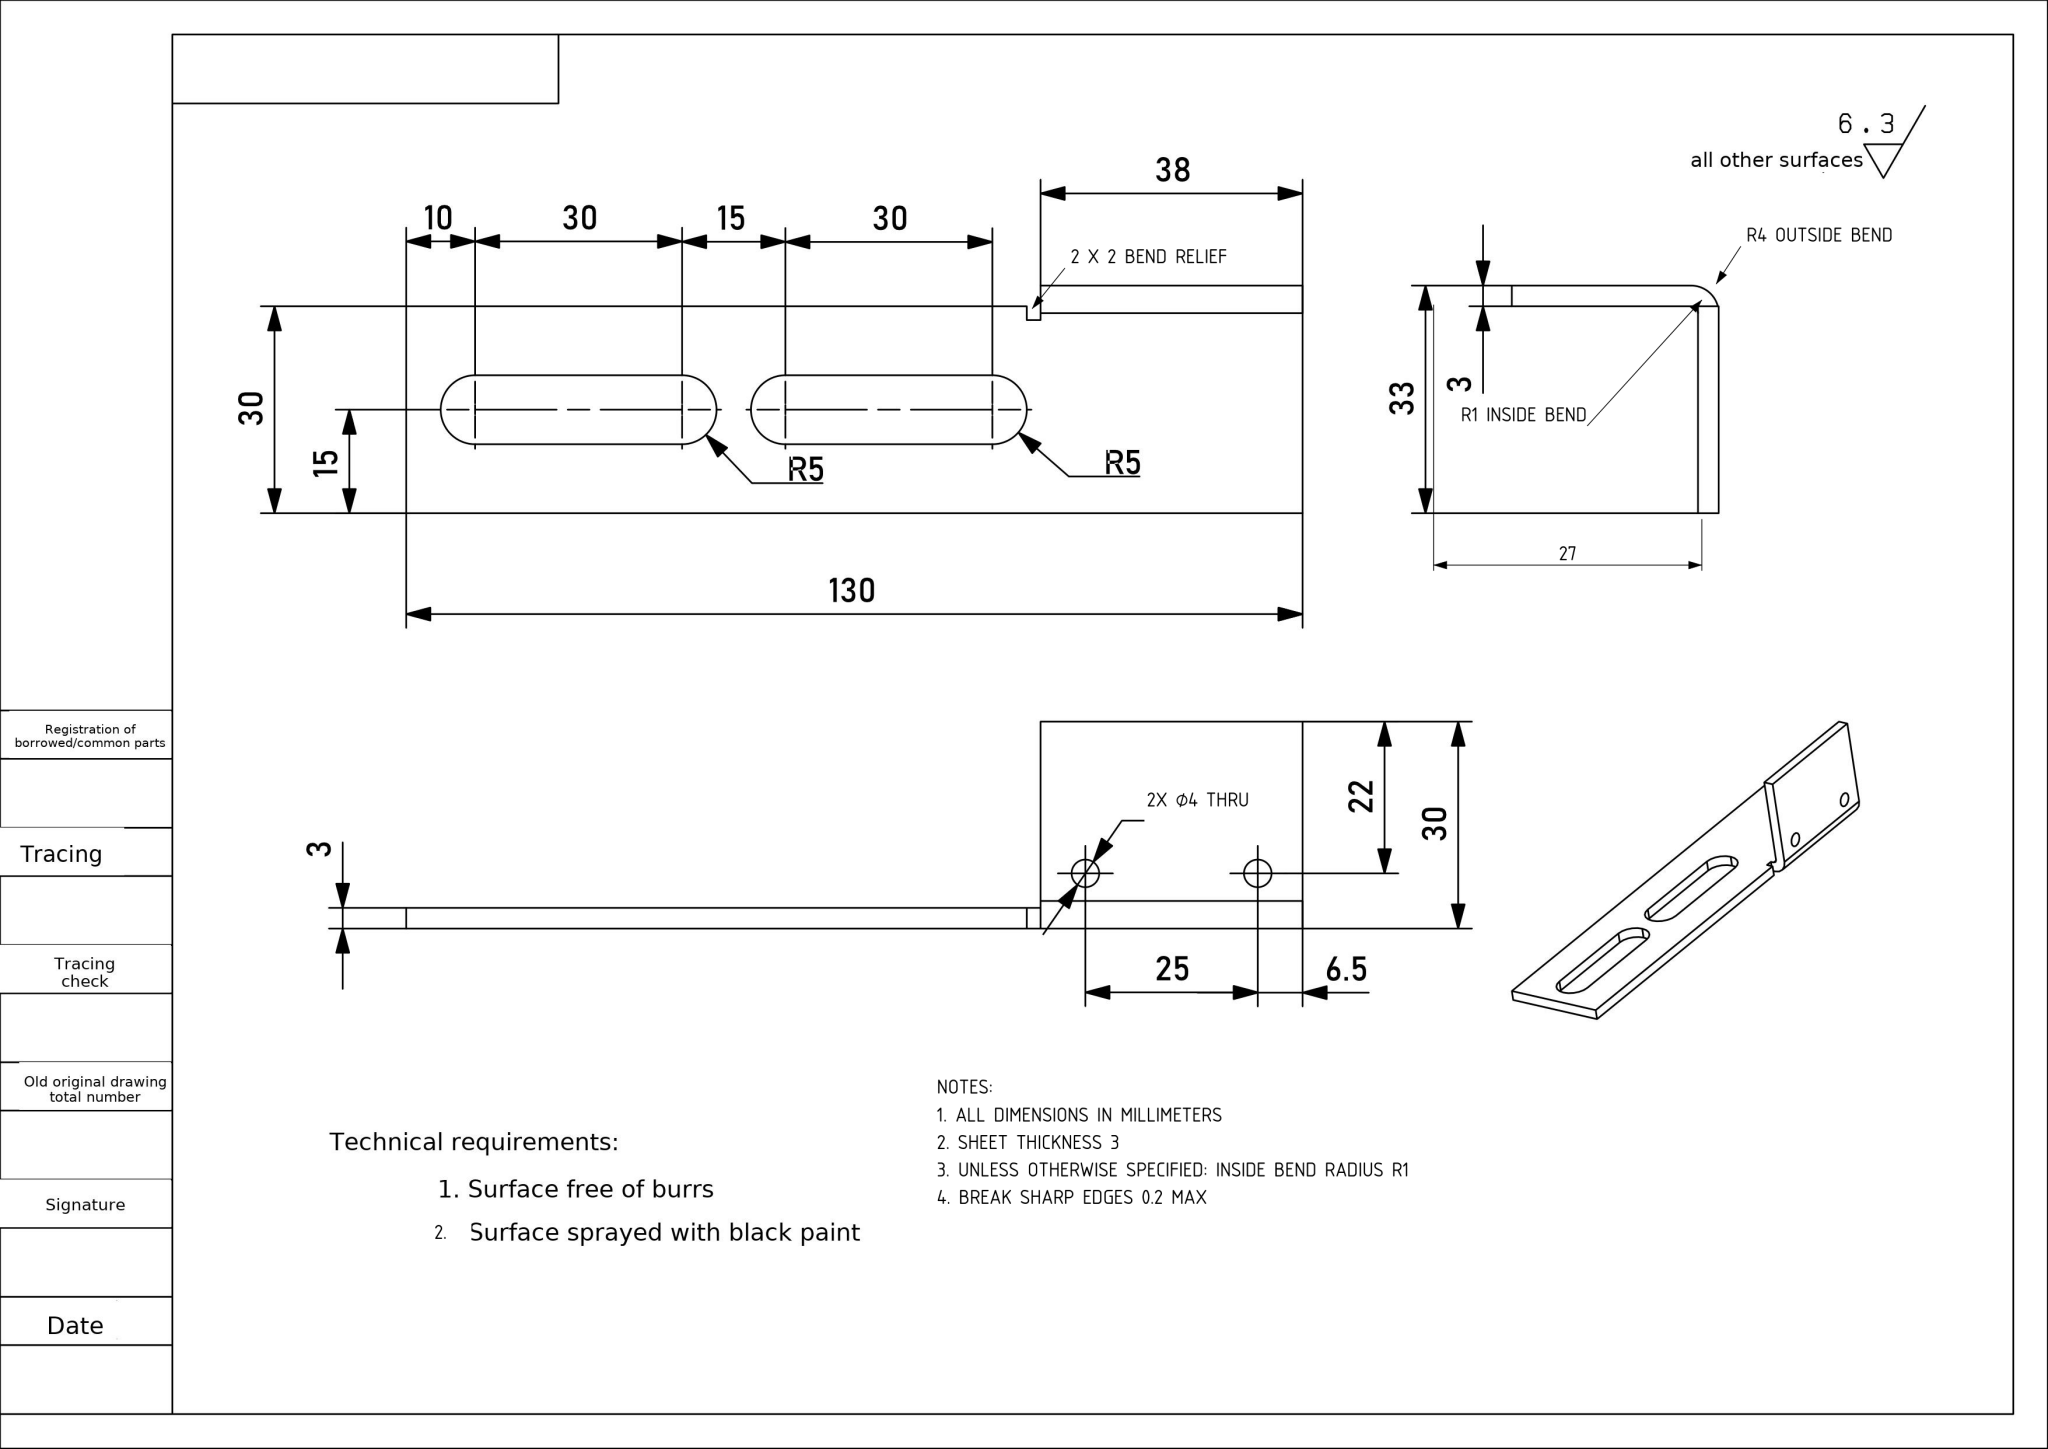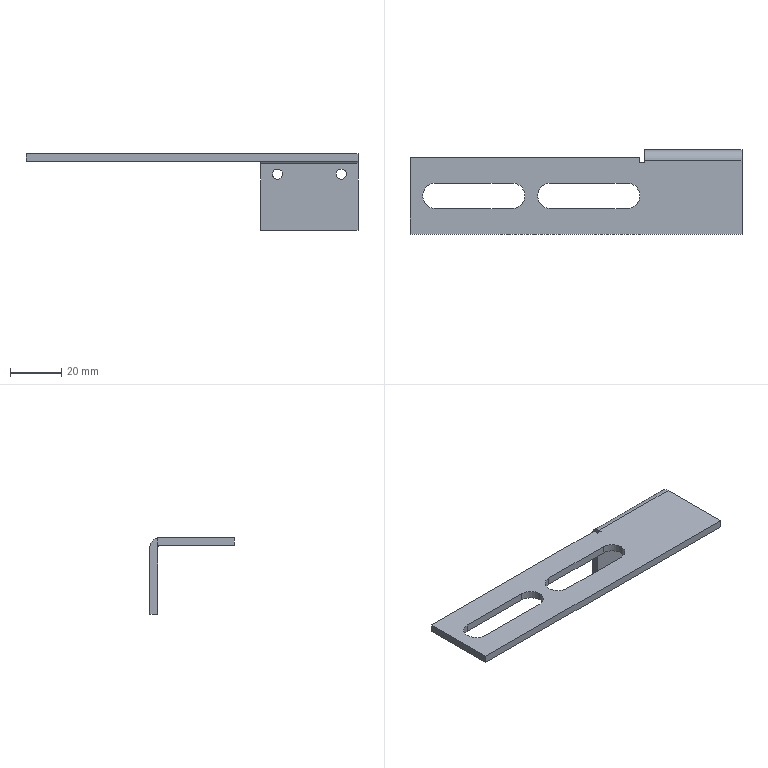Part | NX | mm | 1 solid | 32 faces | box 130 x 33 x 30 mm | volume 12639 mm3 | plane 20 | cylinder 12 | commonest cylinder face diameters 9.98 x8 4 x2 8 x1 2 x1
STEP:
#1=CARTESIAN_POINT('',(0.,0.,0.));
#2=DIRECTION('',(0.,0.,1.));
#3=DIRECTION('',(1.,0.,0.));
#4=AXIS2_PLACEMENT_3D('',#1,#2,#3);
#5=(LENGTH_UNIT()NAMED_UNIT(*)SI_UNIT(.MILLI.,.METRE.));
#6=UNCERTAINTY_MEASURE_WITH_UNIT(LENGTH_MEASURE(0.00002),#5,'','');
#7=(NAMED_UNIT(*)PLANE_ANGLE_UNIT()SI_UNIT($,.RADIAN.));
#8=PLANE_ANGLE_MEASURE_WITH_UNIT(PLANE_ANGLE_MEASURE(0.01745),#7);
#9=DIMENSIONAL_EXPONENTS(0.,0.,0.,0.,0.,0.,0.);
#10=(CONVERSION_BASED_UNIT('',#8)NAMED_UNIT(#9)PLANE_ANGLE_UNIT());
#11=(NAMED_UNIT(*)SI_UNIT($,.STERADIAN.)SOLID_ANGLE_UNIT());
#12=(GEOMETRIC_REPRESENTATION_CONTEXT(3)GLOBAL_UNCERTAINTY_ASSIGNED_CONTEXT((#6))GLOBAL_UNIT_ASSIGNED_CONTEXT((#5,#10,#11))REPRESENTATION_CONTEXT('',''));
#13=SHAPE_REPRESENTATION('',(#4),#12);
#14=CARTESIAN_POINT('',(130.,-30.,0.));
#15=VERTEX_POINT('',#14);
#16=CARTESIAN_POINT('',(130.,-1.,0.));
#17=VERTEX_POINT('',#16);
#18=CARTESIAN_POINT('',(130.,-30.,0.));
#19=DIRECTION('',(0.,1.,0.));
#20=VECTOR('',#19,1.);
#21=LINE('',#18,#20);
#22=EDGE_CURVE('',#15,#17,#21,.T.);
#23=ORIENTED_EDGE('',*,*,#22,.T.);
#24=CARTESIAN_POINT('',(130.,0.,-1.));
#25=VERTEX_POINT('',#24);
#26=CARTESIAN_POINT('',(130.,-1.,-1.));
#27=DIRECTION('',(-1.,0.,0.));
#28=DIRECTION('',(0.,-1.,0.));
#29=AXIS2_PLACEMENT_3D('',#26,#27,#28);
#30=CIRCLE('',#29,1.);
#31=EDGE_CURVE('',#17,#25,#30,.T.);
#32=ORIENTED_EDGE('',*,*,#31,.T.);
#33=CARTESIAN_POINT('',(130.,0.,-27.));
#34=VERTEX_POINT('',#33);
#35=CARTESIAN_POINT('',(130.,0.,-27.));
#36=DIRECTION('',(0.,-0.,1.));
#37=VECTOR('',#36,1.);
#38=LINE('',#35,#37);
#39=EDGE_CURVE('',#34,#25,#38,.T.);
#40=ORIENTED_EDGE('',*,*,#39,.F.);
#41=CARTESIAN_POINT('',(130.,3.,-27.));
#42=VERTEX_POINT('',#41);
#43=CARTESIAN_POINT('',(130.,3.,-27.));
#44=DIRECTION('',(-0.,-1.,-0.));
#45=VECTOR('',#44,1.);
#46=LINE('',#43,#45);
#47=EDGE_CURVE('',#42,#34,#46,.T.);
#48=ORIENTED_EDGE('',*,*,#47,.F.);
#49=CARTESIAN_POINT('',(130.,3.,-1.));
#50=VERTEX_POINT('',#49);
#51=CARTESIAN_POINT('',(130.,3.,-27.));
#52=DIRECTION('',(0.,-0.,1.));
#53=VECTOR('',#52,1.);
#54=LINE('',#51,#53);
#55=EDGE_CURVE('',#42,#50,#54,.T.);
#56=ORIENTED_EDGE('',*,*,#55,.T.);
#57=CARTESIAN_POINT('',(130.,-1.,3.));
#58=VERTEX_POINT('',#57);
#59=CARTESIAN_POINT('',(130.,-1.,-1.));
#60=DIRECTION('',(-1.,0.,0.));
#61=DIRECTION('',(0.,0.,-1.));
#62=AXIS2_PLACEMENT_3D('',#59,#60,#61);
#63=CIRCLE('',#62,4.);
#64=EDGE_CURVE('',#58,#50,#63,.T.);
#65=ORIENTED_EDGE('',*,*,#64,.F.);
#66=CARTESIAN_POINT('',(130.,-30.,3.));
#67=VERTEX_POINT('',#66);
#68=CARTESIAN_POINT('',(130.,-30.,3.));
#69=DIRECTION('',(0.,1.,0.));
#70=VECTOR('',#69,1.);
#71=LINE('',#68,#70);
#72=EDGE_CURVE('',#67,#58,#71,.T.);
#73=ORIENTED_EDGE('',*,*,#72,.F.);
#74=CARTESIAN_POINT('',(130.,-30.,3.));
#75=DIRECTION('',(0.,0.,-1.));
#76=VECTOR('',#75,1.);
#77=LINE('',#74,#76);
#78=EDGE_CURVE('',#67,#15,#77,.T.);
#79=ORIENTED_EDGE('',*,*,#78,.T.);
#80=EDGE_LOOP('',(#23,#32,#40,#48,#56,#65,#73,#79));
#81=FACE_OUTER_BOUND('',#80,.T.);
#82=CARTESIAN_POINT('',(130.,-30.,3.));
#83=DIRECTION('',(-1.,0.,0.));
#84=DIRECTION('',(0.,0.,1.));
#85=AXIS2_PLACEMENT_3D('',#82,#83,#84);
#86=PLANE('',#85);
#87=ADVANCED_FACE('',(#81),#86,.F.);
#88=CARTESIAN_POINT('',(92.,-1.,3.));
#89=VERTEX_POINT('',#88);
#90=CARTESIAN_POINT('',(92.,-2.,3.));
#91=VERTEX_POINT('',#90);
#92=CARTESIAN_POINT('',(92.,0.,3.));
#93=DIRECTION('',(0.,-1.,0.));
#94=VECTOR('',#93,1.);
#95=LINE('',#92,#94);
#96=EDGE_CURVE('',#89,#91,#95,.T.);
#97=ORIENTED_EDGE('',*,*,#96,.F.);
#98=CARTESIAN_POINT('',(92.,3.,-1.));
#99=VERTEX_POINT('',#98);
#100=CARTESIAN_POINT('',(92.,-1.,-1.));
#101=DIRECTION('',(1.,-0.,0.));
#102=DIRECTION('',(0.,0.,-1.));
#103=AXIS2_PLACEMENT_3D('',#100,#101,#102);
#104=CIRCLE('',#103,4.);
#105=EDGE_CURVE('',#99,#89,#104,.T.);
#106=ORIENTED_EDGE('',*,*,#105,.F.);
#107=CARTESIAN_POINT('',(92.,3.,-27.));
#108=VERTEX_POINT('',#107);
#109=CARTESIAN_POINT('',(92.,3.,0.5629));
#110=DIRECTION('',(0.,0.,-1.));
#111=VECTOR('',#110,1.);
#112=LINE('',#109,#111);
#113=EDGE_CURVE('',#99,#108,#112,.T.);
#114=ORIENTED_EDGE('',*,*,#113,.T.);
#115=CARTESIAN_POINT('',(92.,0.,-27.));
#116=VERTEX_POINT('',#115);
#117=CARTESIAN_POINT('',(92.,3.,-27.));
#118=DIRECTION('',(-0.,-1.,-0.));
#119=VECTOR('',#118,1.);
#120=LINE('',#117,#119);
#121=EDGE_CURVE('',#108,#116,#120,.T.);
#122=ORIENTED_EDGE('',*,*,#121,.T.);
#123=CARTESIAN_POINT('',(92.,0.,-1.));
#124=VERTEX_POINT('',#123);
#125=CARTESIAN_POINT('',(92.,-0.,0.5629));
#126=DIRECTION('',(0.,0.,-1.));
#127=VECTOR('',#126,1.);
#128=LINE('',#125,#127);
#129=EDGE_CURVE('',#124,#116,#128,.T.);
#130=ORIENTED_EDGE('',*,*,#129,.F.);
#131=CARTESIAN_POINT('',(92.,-1.,0.));
#132=VERTEX_POINT('',#131);
#133=CARTESIAN_POINT('',(92.,-1.,-1.));
#134=DIRECTION('',(1.,-0.,0.));
#135=DIRECTION('',(0.,-1.,0.));
#136=AXIS2_PLACEMENT_3D('',#133,#134,#135);
#137=CIRCLE('',#136,1.);
#138=EDGE_CURVE('',#124,#132,#137,.T.);
#139=ORIENTED_EDGE('',*,*,#138,.T.);
#140=CARTESIAN_POINT('',(92.,-2.,0.));
#141=VERTEX_POINT('',#140);
#142=CARTESIAN_POINT('',(92.,-2.,0.));
#143=DIRECTION('',(0.,-1.,0.));
#144=VECTOR('',#143,1.);
#145=LINE('',#142,#144);
#146=EDGE_CURVE('',#132,#141,#145,.T.);
#147=ORIENTED_EDGE('',*,*,#146,.T.);
#148=CARTESIAN_POINT('',(92.,-2.,3.));
#149=DIRECTION('',(0.,0.,1.));
#150=VECTOR('',#149,1.);
#151=LINE('',#148,#150);
#152=EDGE_CURVE('',#141,#91,#151,.T.);
#153=ORIENTED_EDGE('',*,*,#152,.T.);
#154=EDGE_LOOP('',(#97,#106,#114,#122,#130,#139,#147,#153));
#155=FACE_OUTER_BOUND('',#154,.T.);
#156=CARTESIAN_POINT('',(92.,0.,3.));
#157=DIRECTION('',(1.,0.,0.));
#158=DIRECTION('',(0.,-1.,0.));
#159=AXIS2_PLACEMENT_3D('',#156,#157,#158);
#160=PLANE('',#159);
#161=ADVANCED_FACE('',(#155),#160,.F.);
#162=CARTESIAN_POINT('',(5.,-15.01,3.));
#163=VERTEX_POINT('',#162);
#164=CARTESIAN_POINT('',(5.,-14.99,3.));
#165=VERTEX_POINT('',#164);
#166=CARTESIAN_POINT('',(5.,-15.01,3.));
#167=DIRECTION('',(0.,1.,0.));
#168=VECTOR('',#167,1.);
#169=LINE('',#166,#168);
#170=EDGE_CURVE('',#163,#165,#169,.T.);
#171=ORIENTED_EDGE('',*,*,#170,.T.);
#172=CARTESIAN_POINT('',(9.99,-10.,3.));
#173=VERTEX_POINT('',#172);
#174=CARTESIAN_POINT('',(9.99,-14.99,3.));
#175=DIRECTION('',(0.,0.,-1.));
#176=DIRECTION('',(1.,0.,0.));
#177=AXIS2_PLACEMENT_3D('',#174,#175,#176);
#178=CIRCLE('',#177,4.99);
#179=EDGE_CURVE('',#165,#173,#178,.T.);
#180=ORIENTED_EDGE('',*,*,#179,.T.);
#181=CARTESIAN_POINT('',(40.01,-10.,3.));
#182=VERTEX_POINT('',#181);
#183=CARTESIAN_POINT('',(9.99,-10.,3.));
#184=DIRECTION('',(1.,-0.,0.));
#185=VECTOR('',#184,1.);
#186=LINE('',#183,#185);
#187=EDGE_CURVE('',#173,#182,#186,.T.);
#188=ORIENTED_EDGE('',*,*,#187,.T.);
#189=CARTESIAN_POINT('',(45.,-14.99,3.));
#190=VERTEX_POINT('',#189);
#191=CARTESIAN_POINT('',(40.01,-14.99,3.));
#192=DIRECTION('',(0.,0.,-1.));
#193=DIRECTION('',(1.,0.,0.));
#194=AXIS2_PLACEMENT_3D('',#191,#192,#193);
#195=CIRCLE('',#194,4.99);
#196=EDGE_CURVE('',#182,#190,#195,.T.);
#197=ORIENTED_EDGE('',*,*,#196,.T.);
#198=CARTESIAN_POINT('',(45.,-15.01,3.));
#199=VERTEX_POINT('',#198);
#200=CARTESIAN_POINT('',(45.,-14.99,3.));
#201=DIRECTION('',(0.,-1.,0.));
#202=VECTOR('',#201,1.);
#203=LINE('',#200,#202);
#204=EDGE_CURVE('',#190,#199,#203,.T.);
#205=ORIENTED_EDGE('',*,*,#204,.T.);
#206=CARTESIAN_POINT('',(40.01,-20.,3.));
#207=VERTEX_POINT('',#206);
#208=CARTESIAN_POINT('',(40.01,-15.01,3.));
#209=DIRECTION('',(0.,0.,-1.));
#210=DIRECTION('',(1.,0.,0.));
#211=AXIS2_PLACEMENT_3D('',#208,#209,#210);
#212=CIRCLE('',#211,4.99);
#213=EDGE_CURVE('',#199,#207,#212,.T.);
#214=ORIENTED_EDGE('',*,*,#213,.T.);
#215=CARTESIAN_POINT('',(9.99,-20.,3.));
#216=VERTEX_POINT('',#215);
#217=CARTESIAN_POINT('',(40.01,-20.,3.));
#218=DIRECTION('',(-1.,-0.,0.));
#219=VECTOR('',#218,1.);
#220=LINE('',#217,#219);
#221=EDGE_CURVE('',#207,#216,#220,.T.);
#222=ORIENTED_EDGE('',*,*,#221,.T.);
#223=CARTESIAN_POINT('',(9.99,-15.01,3.));
#224=DIRECTION('',(0.,0.,-1.));
#225=DIRECTION('',(1.,0.,0.));
#226=AXIS2_PLACEMENT_3D('',#223,#224,#225);
#227=CIRCLE('',#226,4.99);
#228=EDGE_CURVE('',#216,#163,#227,.T.);
#229=ORIENTED_EDGE('',*,*,#228,.T.);
#230=EDGE_LOOP('',(#171,#180,#188,#197,#205,#214,#222,#229));
#231=FACE_BOUND('',#230,.T.);
#232=CARTESIAN_POINT('',(50.,-15.01,3.));
#233=VERTEX_POINT('',#232);
#234=CARTESIAN_POINT('',(50.,-14.99,3.));
#235=VERTEX_POINT('',#234);
#236=CARTESIAN_POINT('',(50.,-15.01,3.));
#237=DIRECTION('',(0.,1.,0.));
#238=VECTOR('',#237,1.);
#239=LINE('',#236,#238);
#240=EDGE_CURVE('',#233,#235,#239,.T.);
#241=ORIENTED_EDGE('',*,*,#240,.T.);
#242=CARTESIAN_POINT('',(54.99,-10.,3.));
#243=VERTEX_POINT('',#242);
#244=CARTESIAN_POINT('',(54.99,-14.99,3.));
#245=DIRECTION('',(0.,0.,-1.));
#246=DIRECTION('',(1.,0.,0.));
#247=AXIS2_PLACEMENT_3D('',#244,#245,#246);
#248=CIRCLE('',#247,4.99);
#249=EDGE_CURVE('',#235,#243,#248,.T.);
#250=ORIENTED_EDGE('',*,*,#249,.T.);
#251=CARTESIAN_POINT('',(85.01,-10.,3.));
#252=VERTEX_POINT('',#251);
#253=CARTESIAN_POINT('',(54.99,-10.,3.));
#254=DIRECTION('',(1.,-0.,0.));
#255=VECTOR('',#254,1.);
#256=LINE('',#253,#255);
#257=EDGE_CURVE('',#243,#252,#256,.T.);
#258=ORIENTED_EDGE('',*,*,#257,.T.);
#259=CARTESIAN_POINT('',(90.,-14.99,3.));
#260=VERTEX_POINT('',#259);
#261=CARTESIAN_POINT('',(85.01,-14.99,3.));
#262=DIRECTION('',(0.,0.,-1.));
#263=DIRECTION('',(1.,0.,0.));
#264=AXIS2_PLACEMENT_3D('',#261,#262,#263);
#265=CIRCLE('',#264,4.99);
#266=EDGE_CURVE('',#252,#260,#265,.T.);
#267=ORIENTED_EDGE('',*,*,#266,.T.);
#268=CARTESIAN_POINT('',(90.,-15.01,3.));
#269=VERTEX_POINT('',#268);
#270=CARTESIAN_POINT('',(90.,-14.99,3.));
#271=DIRECTION('',(0.,-1.,0.));
#272=VECTOR('',#271,1.);
#273=LINE('',#270,#272);
#274=EDGE_CURVE('',#260,#269,#273,.T.);
#275=ORIENTED_EDGE('',*,*,#274,.T.);
#276=CARTESIAN_POINT('',(85.01,-20.,3.));
#277=VERTEX_POINT('',#276);
#278=CARTESIAN_POINT('',(85.01,-15.01,3.));
#279=DIRECTION('',(0.,0.,-1.));
#280=DIRECTION('',(1.,0.,0.));
#281=AXIS2_PLACEMENT_3D('',#278,#279,#280);
#282=CIRCLE('',#281,4.99);
#283=EDGE_CURVE('',#269,#277,#282,.T.);
#284=ORIENTED_EDGE('',*,*,#283,.T.);
#285=CARTESIAN_POINT('',(54.99,-20.,3.));
#286=VERTEX_POINT('',#285);
#287=CARTESIAN_POINT('',(85.01,-20.,3.));
#288=DIRECTION('',(-1.,0.,0.));
#289=VECTOR('',#288,1.);
#290=LINE('',#287,#289);
#291=EDGE_CURVE('',#277,#286,#290,.T.);
#292=ORIENTED_EDGE('',*,*,#291,.T.);
#293=CARTESIAN_POINT('',(54.99,-15.01,3.));
#294=DIRECTION('',(0.,0.,-1.));
#295=DIRECTION('',(1.,0.,0.));
#296=AXIS2_PLACEMENT_3D('',#293,#294,#295);
#297=CIRCLE('',#296,4.99);
#298=EDGE_CURVE('',#286,#233,#297,.T.);
#299=ORIENTED_EDGE('',*,*,#298,.T.);
#300=EDGE_LOOP('',(#241,#250,#258,#267,#275,#284,#292,#299));
#301=FACE_BOUND('',#300,.T.);
#302=ORIENTED_EDGE('',*,*,#72,.T.);
#303=CARTESIAN_POINT('',(130.,-1.,3.));
#304=DIRECTION('',(-1.,0.,0.));
#305=VECTOR('',#304,1.);
#306=LINE('',#303,#305);
#307=EDGE_CURVE('',#58,#89,#306,.T.);
#308=ORIENTED_EDGE('',*,*,#307,.T.);
#309=ORIENTED_EDGE('',*,*,#96,.T.);
#310=CARTESIAN_POINT('',(90.,-2.,3.));
#311=VERTEX_POINT('',#310);
#312=CARTESIAN_POINT('',(90.,-2.,3.));
#313=DIRECTION('',(-1.,0.,0.));
#314=VECTOR('',#313,1.);
#315=LINE('',#312,#314);
#316=EDGE_CURVE('',#91,#311,#315,.T.);
#317=ORIENTED_EDGE('',*,*,#316,.T.);
#318=CARTESIAN_POINT('',(90.,0.,3.));
#319=VERTEX_POINT('',#318);
#320=CARTESIAN_POINT('',(90.,0.,3.));
#321=DIRECTION('',(0.,1.,0.));
#322=VECTOR('',#321,1.);
#323=LINE('',#320,#322);
#324=EDGE_CURVE('',#311,#319,#323,.T.);
#325=ORIENTED_EDGE('',*,*,#324,.T.);
#326=CARTESIAN_POINT('',(0.,0.,3.));
#327=VERTEX_POINT('',#326);
#328=CARTESIAN_POINT('',(130.,0.,3.));
#329=DIRECTION('',(-1.,0.,0.));
#330=VECTOR('',#329,1.);
#331=LINE('',#328,#330);
#332=EDGE_CURVE('',#319,#327,#331,.T.);
#333=ORIENTED_EDGE('',*,*,#332,.T.);
#334=CARTESIAN_POINT('',(0.,-30.,3.));
#335=VERTEX_POINT('',#334);
#336=CARTESIAN_POINT('',(0.,0.,3.));
#337=DIRECTION('',(0.,-1.,0.));
#338=VECTOR('',#337,1.);
#339=LINE('',#336,#338);
#340=EDGE_CURVE('',#327,#335,#339,.T.);
#341=ORIENTED_EDGE('',*,*,#340,.T.);
#342=CARTESIAN_POINT('',(0.,-30.,3.));
#343=DIRECTION('',(1.,0.,0.));
#344=VECTOR('',#343,1.);
#345=LINE('',#342,#344);
#346=EDGE_CURVE('',#335,#67,#345,.T.);
#347=ORIENTED_EDGE('',*,*,#346,.T.);
#348=EDGE_LOOP('',(#302,#308,#309,#317,#325,#333,#341,#347));
#349=FACE_BOUND('',#348,.T.);
#350=CARTESIAN_POINT('',(9.99,-14.99,3.));
#351=DIRECTION('',(0.,0.,-1.));
#352=DIRECTION('',(-1.,0.,0.));
#353=AXIS2_PLACEMENT_3D('',#350,#351,#352);
#354=PLANE('',#353);
#355=ADVANCED_FACE('',(#231,#301,#349),#354,.F.);
#356=ORIENTED_EDGE('',*,*,#332,.F.);
#357=CARTESIAN_POINT('',(90.,0.,0.));
#358=VERTEX_POINT('',#357);
#359=CARTESIAN_POINT('',(90.,0.,3.));
#360=DIRECTION('',(0.,0.,1.));
#361=VECTOR('',#360,1.);
#362=LINE('',#359,#361);
#363=EDGE_CURVE('',#358,#319,#362,.T.);
#364=ORIENTED_EDGE('',*,*,#363,.F.);
#365=CARTESIAN_POINT('',(0.,0.,0.));
#366=VERTEX_POINT('',#365);
#367=CARTESIAN_POINT('',(130.,0.,0.));
#368=DIRECTION('',(-1.,0.,0.));
#369=VECTOR('',#368,1.);
#370=LINE('',#367,#369);
#371=EDGE_CURVE('',#358,#366,#370,.T.);
#372=ORIENTED_EDGE('',*,*,#371,.T.);
#373=CARTESIAN_POINT('',(0.,0.,3.));
#374=DIRECTION('',(0.,0.,-1.));
#375=VECTOR('',#374,1.);
#376=LINE('',#373,#375);
#377=EDGE_CURVE('',#327,#366,#376,.T.);
#378=ORIENTED_EDGE('',*,*,#377,.F.);
#379=EDGE_LOOP('',(#356,#364,#372,#378));
#380=FACE_OUTER_BOUND('',#379,.T.);
#381=CARTESIAN_POINT('',(130.,0.,3.));
#382=DIRECTION('',(0.,-1.,0.));
#383=DIRECTION('',(0.,0.,-1.));
#384=AXIS2_PLACEMENT_3D('',#381,#382,#383);
#385=PLANE('',#384);
#386=ADVANCED_FACE('',(#380),#385,.F.);
#387=CARTESIAN_POINT('',(50.,-15.01,0.));
#388=VERTEX_POINT('',#387);
#389=CARTESIAN_POINT('',(50.,-14.99,0.));
#390=VERTEX_POINT('',#389);
#391=CARTESIAN_POINT('',(50.,-15.01,0.));
#392=DIRECTION('',(0.,1.,0.));
#393=VECTOR('',#392,1.);
#394=LINE('',#391,#393);
#395=EDGE_CURVE('',#388,#390,#394,.T.);
#396=ORIENTED_EDGE('',*,*,#395,.T.);
#397=CARTESIAN_POINT('',(50.,-14.99,3.));
#398=DIRECTION('',(0.,0.,-1.));
#399=VECTOR('',#398,1.);
#400=LINE('',#397,#399);
#401=EDGE_CURVE('',#235,#390,#400,.T.);
#402=ORIENTED_EDGE('',*,*,#401,.F.);
#403=ORIENTED_EDGE('',*,*,#240,.F.);
#404=CARTESIAN_POINT('',(50.,-15.01,3.));
#405=DIRECTION('',(0.,0.,-1.));
#406=VECTOR('',#405,1.);
#407=LINE('',#404,#406);
#408=EDGE_CURVE('',#233,#388,#407,.T.);
#409=ORIENTED_EDGE('',*,*,#408,.T.);
#410=EDGE_LOOP('',(#396,#402,#403,#409));
#411=FACE_OUTER_BOUND('',#410,.T.);
#412=CARTESIAN_POINT('',(50.,-15.01,3.));
#413=DIRECTION('',(-1.,0.,0.));
#414=DIRECTION('',(0.,0.,1.));
#415=AXIS2_PLACEMENT_3D('',#412,#413,#414);
#416=PLANE('',#415);
#417=ADVANCED_FACE('',(#411),#416,.F.);
#418=CARTESIAN_POINT('',(54.99,-10.,0.));
#419=VERTEX_POINT('',#418);
#420=CARTESIAN_POINT('',(54.99,-14.99,0.));
#421=DIRECTION('',(0.,0.,-1.));
#422=DIRECTION('',(1.,0.,0.));
#423=AXIS2_PLACEMENT_3D('',#420,#421,#422);
#424=CIRCLE('',#423,4.99);
#425=EDGE_CURVE('',#390,#419,#424,.T.);
#426=ORIENTED_EDGE('',*,*,#425,.T.);
#427=CARTESIAN_POINT('',(54.99,-10.,3.));
#428=DIRECTION('',(0.,0.,-1.));
#429=VECTOR('',#428,1.);
#430=LINE('',#427,#429);
#431=EDGE_CURVE('',#243,#419,#430,.T.);
#432=ORIENTED_EDGE('',*,*,#431,.F.);
#433=ORIENTED_EDGE('',*,*,#249,.F.);
#434=ORIENTED_EDGE('',*,*,#401,.T.);
#435=EDGE_LOOP('',(#426,#432,#433,#434));
#436=FACE_OUTER_BOUND('',#435,.T.);
#437=CARTESIAN_POINT('',(54.99,-14.99,3.));
#438=DIRECTION('',(0.,0.,-1.));
#439=DIRECTION('',(-1.,0.,0.));
#440=AXIS2_PLACEMENT_3D('',#437,#438,#439);
#441=CYLINDRICAL_SURFACE('',#440,4.99);
#442=ADVANCED_FACE('',(#436),#441,.F.);
#443=CARTESIAN_POINT('',(85.01,-10.,0.));
#444=VERTEX_POINT('',#443);
#445=CARTESIAN_POINT('',(54.99,-10.,0.));
#446=DIRECTION('',(1.,-0.,0.));
#447=VECTOR('',#446,1.);
#448=LINE('',#445,#447);
#449=EDGE_CURVE('',#419,#444,#448,.T.);
#450=ORIENTED_EDGE('',*,*,#449,.T.);
#451=CARTESIAN_POINT('',(85.01,-10.,3.));
#452=DIRECTION('',(0.,0.,-1.));
#453=VECTOR('',#452,1.);
#454=LINE('',#451,#453);
#455=EDGE_CURVE('',#252,#444,#454,.T.);
#456=ORIENTED_EDGE('',*,*,#455,.F.);
#457=ORIENTED_EDGE('',*,*,#257,.F.);
#458=ORIENTED_EDGE('',*,*,#431,.T.);
#459=EDGE_LOOP('',(#450,#456,#457,#458));
#460=FACE_OUTER_BOUND('',#459,.T.);
#461=CARTESIAN_POINT('',(54.99,-10.,3.));
#462=DIRECTION('',(0.,1.,0.));
#463=DIRECTION('',(-1.,0.,0.));
#464=AXIS2_PLACEMENT_3D('',#461,#462,#463);
#465=PLANE('',#464);
#466=ADVANCED_FACE('',(#460),#465,.F.);
#467=CARTESIAN_POINT('',(90.,-14.99,0.));
#468=VERTEX_POINT('',#467);
#469=CARTESIAN_POINT('',(85.01,-14.99,0.));
#470=DIRECTION('',(0.,0.,-1.));
#471=DIRECTION('',(1.,0.,0.));
#472=AXIS2_PLACEMENT_3D('',#469,#470,#471);
#473=CIRCLE('',#472,4.99);
#474=EDGE_CURVE('',#444,#468,#473,.T.);
#475=ORIENTED_EDGE('',*,*,#474,.T.);
#476=CARTESIAN_POINT('',(90.,-14.99,3.));
#477=DIRECTION('',(0.,0.,-1.));
#478=VECTOR('',#477,1.);
#479=LINE('',#476,#478);
#480=EDGE_CURVE('',#260,#468,#479,.T.);
#481=ORIENTED_EDGE('',*,*,#480,.F.);
#482=ORIENTED_EDGE('',*,*,#266,.F.);
#483=ORIENTED_EDGE('',*,*,#455,.T.);
#484=EDGE_LOOP('',(#475,#481,#482,#483));
#485=FACE_OUTER_BOUND('',#484,.T.);
#486=CARTESIAN_POINT('',(85.01,-14.99,3.));
#487=DIRECTION('',(0.,0.,-1.));
#488=DIRECTION('',(-1.,0.,0.));
#489=AXIS2_PLACEMENT_3D('',#486,#487,#488);
#490=CYLINDRICAL_SURFACE('',#489,4.99);
#491=ADVANCED_FACE('',(#485),#490,.F.);
#492=CARTESIAN_POINT('',(90.,-15.01,0.));
#493=VERTEX_POINT('',#492);
#494=CARTESIAN_POINT('',(90.,-14.99,0.));
#495=DIRECTION('',(0.,-1.,0.));
#496=VECTOR('',#495,1.);
#497=LINE('',#494,#496);
#498=EDGE_CURVE('',#468,#493,#497,.T.);
#499=ORIENTED_EDGE('',*,*,#498,.T.);
#500=CARTESIAN_POINT('',(90.,-15.01,3.));
#501=DIRECTION('',(0.,0.,-1.));
#502=VECTOR('',#501,1.);
#503=LINE('',#500,#502);
#504=EDGE_CURVE('',#269,#493,#503,.T.);
#505=ORIENTED_EDGE('',*,*,#504,.F.);
#506=ORIENTED_EDGE('',*,*,#274,.F.);
#507=ORIENTED_EDGE('',*,*,#480,.T.);
#508=EDGE_LOOP('',(#499,#505,#506,#507));
#509=FACE_OUTER_BOUND('',#508,.T.);
#510=CARTESIAN_POINT('',(90.,-14.99,3.));
#511=DIRECTION('',(1.,0.,0.));
#512=DIRECTION('',(0.,0.,-1.));
#513=AXIS2_PLACEMENT_3D('',#510,#511,#512);
#514=PLANE('',#513);
#515=ADVANCED_FACE('',(#509),#514,.F.);
#516=CARTESIAN_POINT('',(85.01,-20.,0.));
#517=VERTEX_POINT('',#516);
#518=CARTESIAN_POINT('',(85.01,-15.01,0.));
#519=DIRECTION('',(0.,0.,-1.));
#520=DIRECTION('',(1.,0.,0.));
#521=AXIS2_PLACEMENT_3D('',#518,#519,#520);
#522=CIRCLE('',#521,4.99);
#523=EDGE_CURVE('',#493,#517,#522,.T.);
#524=ORIENTED_EDGE('',*,*,#523,.T.);
#525=CARTESIAN_POINT('',(85.01,-20.,3.));
#526=DIRECTION('',(0.,0.,-1.));
#527=VECTOR('',#526,1.);
#528=LINE('',#525,#527);
#529=EDGE_CURVE('',#277,#517,#528,.T.);
#530=ORIENTED_EDGE('',*,*,#529,.F.);
#531=ORIENTED_EDGE('',*,*,#283,.F.);
#532=ORIENTED_EDGE('',*,*,#504,.T.);
#533=EDGE_LOOP('',(#524,#530,#531,#532));
#534=FACE_OUTER_BOUND('',#533,.T.);
#535=CARTESIAN_POINT('',(85.01,-15.01,3.));
#536=DIRECTION('',(0.,0.,-1.));
#537=DIRECTION('',(-1.,0.,0.));
#538=AXIS2_PLACEMENT_3D('',#535,#536,#537);
#539=CYLINDRICAL_SURFACE('',#538,4.99);
#540=ADVANCED_FACE('',(#534),#539,.F.);
#541=CARTESIAN_POINT('',(54.99,-20.,0.));
#542=VERTEX_POINT('',#541);
#543=CARTESIAN_POINT('',(85.01,-20.,0.));
#544=DIRECTION('',(-1.,0.,0.));
#545=VECTOR('',#544,1.);
#546=LINE('',#543,#545);
#547=EDGE_CURVE('',#517,#542,#546,.T.);
#548=ORIENTED_EDGE('',*,*,#547,.T.);
#549=CARTESIAN_POINT('',(54.99,-20.,3.));
#550=DIRECTION('',(0.,0.,-1.));
#551=VECTOR('',#550,1.);
#552=LINE('',#549,#551);
#553=EDGE_CURVE('',#286,#542,#552,.T.);
#554=ORIENTED_EDGE('',*,*,#553,.F.);
#555=ORIENTED_EDGE('',*,*,#291,.F.);
#556=ORIENTED_EDGE('',*,*,#529,.T.);
#557=EDGE_LOOP('',(#548,#554,#555,#556));
#558=FACE_OUTER_BOUND('',#557,.T.);
#559=CARTESIAN_POINT('',(85.01,-20.,3.));
#560=DIRECTION('',(0.,-1.,0.));
#561=DIRECTION('',(0.,0.,-1.));
#562=AXIS2_PLACEMENT_3D('',#559,#560,#561);
#563=PLANE('',#562);
#564=ADVANCED_FACE('',(#558),#563,.F.);
#565=CARTESIAN_POINT('',(5.,-15.01,0.));
#566=VERTEX_POINT('',#565);
#567=CARTESIAN_POINT('',(5.,-14.99,0.));
#568=VERTEX_POINT('',#567);
#569=CARTESIAN_POINT('',(5.,-15.01,0.));
#570=DIRECTION('',(0.,1.,0.));
#571=VECTOR('',#570,1.);
#572=LINE('',#569,#571);
#573=EDGE_CURVE('',#566,#568,#572,.T.);
#574=ORIENTED_EDGE('',*,*,#573,.T.);
#575=CARTESIAN_POINT('',(5.,-14.99,3.));
#576=DIRECTION('',(0.,0.,-1.));
#577=VECTOR('',#576,1.);
#578=LINE('',#575,#577);
#579=EDGE_CURVE('',#165,#568,#578,.T.);
#580=ORIENTED_EDGE('',*,*,#579,.F.);
#581=ORIENTED_EDGE('',*,*,#170,.F.);
#582=CARTESIAN_POINT('',(5.,-15.01,3.));
#583=DIRECTION('',(0.,0.,-1.));
#584=VECTOR('',#583,1.);
#585=LINE('',#582,#584);
#586=EDGE_CURVE('',#163,#566,#585,.T.);
#587=ORIENTED_EDGE('',*,*,#586,.T.);
#588=EDGE_LOOP('',(#574,#580,#581,#587));
#589=FACE_OUTER_BOUND('',#588,.T.);
#590=CARTESIAN_POINT('',(5.,-15.01,3.));
#591=DIRECTION('',(-1.,0.,0.));
#592=DIRECTION('',(0.,0.,1.));
#593=AXIS2_PLACEMENT_3D('',#590,#591,#592);
#594=PLANE('',#593);
#595=ADVANCED_FACE('',(#589),#594,.F.);
#596=CARTESIAN_POINT('',(9.99,-10.,0.));
#597=VERTEX_POINT('',#596);
#598=CARTESIAN_POINT('',(9.99,-14.99,0.));
#599=DIRECTION('',(0.,0.,-1.));
#600=DIRECTION('',(1.,0.,0.));
#601=AXIS2_PLACEMENT_3D('',#598,#599,#600);
#602=CIRCLE('',#601,4.99);
#603=EDGE_CURVE('',#568,#597,#602,.T.);
#604=ORIENTED_EDGE('',*,*,#603,.T.);
#605=CARTESIAN_POINT('',(9.99,-10.,3.));
#606=DIRECTION('',(0.,0.,-1.));
#607=VECTOR('',#606,1.);
#608=LINE('',#605,#607);
#609=EDGE_CURVE('',#173,#597,#608,.T.);
#610=ORIENTED_EDGE('',*,*,#609,.F.);
#611=ORIENTED_EDGE('',*,*,#179,.F.);
#612=ORIENTED_EDGE('',*,*,#579,.T.);
#613=EDGE_LOOP('',(#604,#610,#611,#612));
#614=FACE_OUTER_BOUND('',#613,.T.);
#615=CARTESIAN_POINT('',(9.99,-14.99,3.));
#616=DIRECTION('',(0.,0.,-1.));
#617=DIRECTION('',(-1.,0.,0.));
#618=AXIS2_PLACEMENT_3D('',#615,#616,#617);
#619=CYLINDRICAL_SURFACE('',#618,4.99);
#620=ADVANCED_FACE('',(#614),#619,.F.);
#621=CARTESIAN_POINT('',(40.01,-10.,0.));
#622=VERTEX_POINT('',#621);
#623=CARTESIAN_POINT('',(9.99,-10.,0.));
#624=DIRECTION('',(1.,-0.,0.));
#625=VECTOR('',#624,1.);
#626=LINE('',#623,#625);
#627=EDGE_CURVE('',#597,#622,#626,.T.);
#628=ORIENTED_EDGE('',*,*,#627,.T.);
#629=CARTESIAN_POINT('',(40.01,-10.,3.));
#630=DIRECTION('',(0.,0.,-1.));
#631=VECTOR('',#630,1.);
#632=LINE('',#629,#631);
#633=EDGE_CURVE('',#182,#622,#632,.T.);
#634=ORIENTED_EDGE('',*,*,#633,.F.);
#635=ORIENTED_EDGE('',*,*,#187,.F.);
#636=ORIENTED_EDGE('',*,*,#609,.T.);
#637=EDGE_LOOP('',(#628,#634,#635,#636));
#638=FACE_OUTER_BOUND('',#637,.T.);
#639=CARTESIAN_POINT('',(9.99,-10.,3.));
#640=DIRECTION('',(0.,1.,0.));
#641=DIRECTION('',(-1.,0.,0.));
#642=AXIS2_PLACEMENT_3D('',#639,#640,#641);
#643=PLANE('',#642);
#644=ADVANCED_FACE('',(#638),#643,.F.);
#645=CARTESIAN_POINT('',(45.,-14.99,0.));
#646=VERTEX_POINT('',#645);
#647=CARTESIAN_POINT('',(40.01,-14.99,0.));
#648=DIRECTION('',(0.,0.,-1.));
#649=DIRECTION('',(1.,0.,0.));
#650=AXIS2_PLACEMENT_3D('',#647,#648,#649);
#651=CIRCLE('',#650,4.99);
#652=EDGE_CURVE('',#622,#646,#651,.T.);
#653=ORIENTED_EDGE('',*,*,#652,.T.);
#654=CARTESIAN_POINT('',(45.,-14.99,3.));
#655=DIRECTION('',(0.,0.,-1.));
#656=VECTOR('',#655,1.);
#657=LINE('',#654,#656);
#658=EDGE_CURVE('',#190,#646,#657,.T.);
#659=ORIENTED_EDGE('',*,*,#658,.F.);
#660=ORIENTED_EDGE('',*,*,#196,.F.);
#661=ORIENTED_EDGE('',*,*,#633,.T.);
#662=EDGE_LOOP('',(#653,#659,#660,#661));
#663=FACE_OUTER_BOUND('',#662,.T.);
#664=CARTESIAN_POINT('',(40.01,-14.99,3.));
#665=DIRECTION('',(0.,0.,-1.));
#666=DIRECTION('',(-1.,0.,0.));
#667=AXIS2_PLACEMENT_3D('',#664,#665,#666);
#668=CYLINDRICAL_SURFACE('',#667,4.99);
#669=ADVANCED_FACE('',(#663),#668,.F.);
#670=CARTESIAN_POINT('',(45.,-15.01,0.));
#671=VERTEX_POINT('',#670);
#672=CARTESIAN_POINT('',(45.,-14.99,0.));
#673=DIRECTION('',(0.,-1.,0.));
#674=VECTOR('',#673,1.);
#675=LINE('',#672,#674);
#676=EDGE_CURVE('',#646,#671,#675,.T.);
#677=ORIENTED_EDGE('',*,*,#676,.T.);
#678=CARTESIAN_POINT('',(45.,-15.01,3.));
#679=DIRECTION('',(0.,0.,-1.));
#680=VECTOR('',#679,1.);
#681=LINE('',#678,#680);
#682=EDGE_CURVE('',#199,#671,#681,.T.);
#683=ORIENTED_EDGE('',*,*,#682,.F.);
#684=ORIENTED_EDGE('',*,*,#204,.F.);
#685=ORIENTED_EDGE('',*,*,#658,.T.);
#686=EDGE_LOOP('',(#677,#683,#684,#685));
#687=FACE_OUTER_BOUND('',#686,.T.);
#688=CARTESIAN_POINT('',(45.,-14.99,3.));
#689=DIRECTION('',(1.,0.,0.));
#690=DIRECTION('',(0.,0.,-1.));
#691=AXIS2_PLACEMENT_3D('',#688,#689,#690);
#692=PLANE('',#691);
#693=ADVANCED_FACE('',(#687),#692,.F.);
#694=CARTESIAN_POINT('',(40.01,-20.,0.));
#695=VERTEX_POINT('',#694);
#696=CARTESIAN_POINT('',(40.01,-15.01,0.));
#697=DIRECTION('',(0.,0.,-1.));
#698=DIRECTION('',(1.,0.,0.));
#699=AXIS2_PLACEMENT_3D('',#696,#697,#698);
#700=CIRCLE('',#699,4.99);
#701=EDGE_CURVE('',#671,#695,#700,.T.);
#702=ORIENTED_EDGE('',*,*,#701,.T.);
#703=CARTESIAN_POINT('',(40.01,-20.,3.));
#704=DIRECTION('',(0.,0.,-1.));
#705=VECTOR('',#704,1.);
#706=LINE('',#703,#705);
#707=EDGE_CURVE('',#207,#695,#706,.T.);
#708=ORIENTED_EDGE('',*,*,#707,.F.);
#709=ORIENTED_EDGE('',*,*,#213,.F.);
#710=ORIENTED_EDGE('',*,*,#682,.T.);
#711=EDGE_LOOP('',(#702,#708,#709,#710));
#712=FACE_OUTER_BOUND('',#711,.T.);
#713=CARTESIAN_POINT('',(40.01,-15.01,3.));
#714=DIRECTION('',(0.,0.,-1.));
#715=DIRECTION('',(-1.,0.,0.));
#716=AXIS2_PLACEMENT_3D('',#713,#714,#715);
#717=CYLINDRICAL_SURFACE('',#716,4.99);
#718=ADVANCED_FACE('',(#712),#717,.F.);
#719=CARTESIAN_POINT('',(9.99,-20.,0.));
#720=VERTEX_POINT('',#719);
#721=CARTESIAN_POINT('',(40.01,-20.,0.));
#722=DIRECTION('',(-1.,-0.,0.));
#723=VECTOR('',#722,1.);
#724=LINE('',#721,#723);
#725=EDGE_CURVE('',#695,#720,#724,.T.);
#726=ORIENTED_EDGE('',*,*,#725,.T.);
#727=CARTESIAN_POINT('',(9.99,-20.,3.));
#728=DIRECTION('',(0.,0.,-1.));
#729=VECTOR('',#728,1.);
#730=LINE('',#727,#729);
#731=EDGE_CURVE('',#216,#720,#730,.T.);
#732=ORIENTED_EDGE('',*,*,#731,.F.);
#733=ORIENTED_EDGE('',*,*,#221,.F.);
#734=ORIENTED_EDGE('',*,*,#707,.T.);
#735=EDGE_LOOP('',(#726,#732,#733,#734));
#736=FACE_OUTER_BOUND('',#735,.T.);
#737=CARTESIAN_POINT('',(40.01,-20.,3.));
#738=DIRECTION('',(0.,-1.,0.));
#739=DIRECTION('',(1.,0.,0.));
#740=AXIS2_PLACEMENT_3D('',#737,#738,#739);
#741=PLANE('',#740);
#742=ADVANCED_FACE('',(#736),#741,.F.);
#743=CARTESIAN_POINT('',(0.,-30.,0.));
#744=VERTEX_POINT('',#743);
#745=CARTESIAN_POINT('',(0.,0.,0.));
#746=DIRECTION('',(0.,-1.,0.));
#747=VECTOR('',#746,1.);
#748=LINE('',#745,#747);
#749=EDGE_CURVE('',#366,#744,#748,.T.);
#750=ORIENTED_EDGE('',*,*,#749,.T.);
#751=CARTESIAN_POINT('',(0.,-30.,3.));
#752=DIRECTION('',(0.,0.,-1.));
#753=VECTOR('',#752,1.);
#754=LINE('',#751,#753);
#755=EDGE_CURVE('',#335,#744,#754,.T.);
#756=ORIENTED_EDGE('',*,*,#755,.F.);
#757=ORIENTED_EDGE('',*,*,#340,.F.);
#758=ORIENTED_EDGE('',*,*,#377,.T.);
#759=EDGE_LOOP('',(#750,#756,#757,#758));
#760=FACE_OUTER_BOUND('',#759,.T.);
#761=CARTESIAN_POINT('',(0.,0.,3.));
#762=DIRECTION('',(1.,0.,0.));
#763=DIRECTION('',(0.,0.,-1.));
#764=AXIS2_PLACEMENT_3D('',#761,#762,#763);
#765=PLANE('',#764);
#766=ADVANCED_FACE('',(#760),#765,.F.);
#767=CARTESIAN_POINT('',(0.,-30.,0.));
#768=DIRECTION('',(1.,0.,0.));
#769=VECTOR('',#768,1.);
#770=LINE('',#767,#769);
#771=EDGE_CURVE('',#744,#15,#770,.T.);
#772=ORIENTED_EDGE('',*,*,#771,.T.);
#773=ORIENTED_EDGE('',*,*,#78,.F.);
#774=ORIENTED_EDGE('',*,*,#346,.F.);
#775=ORIENTED_EDGE('',*,*,#755,.T.);
#776=EDGE_LOOP('',(#772,#773,#774,#775));
#777=FACE_OUTER_BOUND('',#776,.T.);
#778=CARTESIAN_POINT('',(0.,-30.,3.));
#779=DIRECTION('',(0.,1.,0.));
#780=DIRECTION('',(0.,0.,1.));
#781=AXIS2_PLACEMENT_3D('',#778,#779,#780);
#782=PLANE('',#781);
#783=ADVANCED_FACE('',(#777),#782,.F.);
#784=CARTESIAN_POINT('',(9.99,-15.01,0.));
#785=DIRECTION('',(0.,0.,-1.));
#786=DIRECTION('',(1.,0.,0.));
#787=AXIS2_PLACEMENT_3D('',#784,#785,#786);
#788=CIRCLE('',#787,4.99);
#789=EDGE_CURVE('',#720,#566,#788,.T.);
#790=ORIENTED_EDGE('',*,*,#789,.T.);
#791=ORIENTED_EDGE('',*,*,#586,.F.);
#792=ORIENTED_EDGE('',*,*,#228,.F.);
#793=ORIENTED_EDGE('',*,*,#731,.T.);
#794=EDGE_LOOP('',(#790,#791,#792,#793));
#795=FACE_OUTER_BOUND('',#794,.T.);
#796=CARTESIAN_POINT('',(9.99,-15.01,3.));
#797=DIRECTION('',(0.,0.,-1.));
#798=DIRECTION('',(-1.,0.,0.));
#799=AXIS2_PLACEMENT_3D('',#796,#797,#798);
#800=CYLINDRICAL_SURFACE('',#799,4.99);
#801=ADVANCED_FACE('',(#795),#800,.F.);
#802=CARTESIAN_POINT('',(54.99,-15.01,0.));
#803=DIRECTION('',(0.,0.,-1.));
#804=DIRECTION('',(1.,0.,0.));
#805=AXIS2_PLACEMENT_3D('',#802,#803,#804);
#806=CIRCLE('',#805,4.99);
#807=EDGE_CURVE('',#542,#388,#806,.T.);
#808=ORIENTED_EDGE('',*,*,#807,.T.);
#809=ORIENTED_EDGE('',*,*,#408,.F.);
#810=ORIENTED_EDGE('',*,*,#298,.F.);
#811=ORIENTED_EDGE('',*,*,#553,.T.);
#812=EDGE_LOOP('',(#808,#809,#810,#811));
#813=FACE_OUTER_BOUND('',#812,.T.);
#814=CARTESIAN_POINT('',(54.99,-15.01,3.));
#815=DIRECTION('',(0.,0.,-1.));
#816=DIRECTION('',(-1.,0.,0.));
#817=AXIS2_PLACEMENT_3D('',#814,#815,#816);
#818=CYLINDRICAL_SURFACE('',#817,4.99);
#819=ADVANCED_FACE('',(#813),#818,.F.);
#820=CARTESIAN_POINT('',(130.,-1.,0.));
#821=DIRECTION('',(-1.,0.,0.));
#822=VECTOR('',#821,1.);
#823=LINE('',#820,#822);
#824=EDGE_CURVE('',#17,#132,#823,.T.);
#825=ORIENTED_EDGE('',*,*,#824,.F.);
#826=ORIENTED_EDGE('',*,*,#22,.F.);
#827=ORIENTED_EDGE('',*,*,#771,.F.);
#828=ORIENTED_EDGE('',*,*,#749,.F.);
#829=ORIENTED_EDGE('',*,*,#371,.F.);
#830=CARTESIAN_POINT('',(90.,-2.,0.));
#831=VERTEX_POINT('',#830);
#832=CARTESIAN_POINT('',(90.,-2.,0.));
#833=DIRECTION('',(0.,1.,0.));
#834=VECTOR('',#833,1.);
#835=LINE('',#832,#834);
#836=EDGE_CURVE('',#831,#358,#835,.T.);
#837=ORIENTED_EDGE('',*,*,#836,.F.);
#838=CARTESIAN_POINT('',(92.,-2.,0.));
#839=DIRECTION('',(-1.,0.,0.));
#840=VECTOR('',#839,1.);
#841=LINE('',#838,#840);
#842=EDGE_CURVE('',#141,#831,#841,.T.);
#843=ORIENTED_EDGE('',*,*,#842,.F.);
#844=ORIENTED_EDGE('',*,*,#146,.F.);
#845=EDGE_LOOP('',(#825,#826,#827,#828,#829,#837,#843,#844));
#846=FACE_BOUND('',#845,.T.);
#847=ORIENTED_EDGE('',*,*,#573,.F.);
#848=ORIENTED_EDGE('',*,*,#789,.F.);
#849=ORIENTED_EDGE('',*,*,#725,.F.);
#850=ORIENTED_EDGE('',*,*,#701,.F.);
#851=ORIENTED_EDGE('',*,*,#676,.F.);
#852=ORIENTED_EDGE('',*,*,#652,.F.);
#853=ORIENTED_EDGE('',*,*,#627,.F.);
#854=ORIENTED_EDGE('',*,*,#603,.F.);
#855=EDGE_LOOP('',(#847,#848,#849,#850,#851,#852,#853,#854));
#856=FACE_BOUND('',#855,.T.);
#857=ORIENTED_EDGE('',*,*,#395,.F.);
#858=ORIENTED_EDGE('',*,*,#807,.F.);
#859=ORIENTED_EDGE('',*,*,#547,.F.);
#860=ORIENTED_EDGE('',*,*,#523,.F.);
#861=ORIENTED_EDGE('',*,*,#498,.F.);
#862=ORIENTED_EDGE('',*,*,#474,.F.);
#863=ORIENTED_EDGE('',*,*,#449,.F.);
#864=ORIENTED_EDGE('',*,*,#425,.F.);
#865=EDGE_LOOP('',(#857,#858,#859,#860,#861,#862,#863,#864));
#866=FACE_BOUND('',#865,.T.);
#867=CARTESIAN_POINT('',(9.99,-14.99,0.));
#868=DIRECTION('',(0.,0.,-1.));
#869=DIRECTION('',(-1.,0.,0.));
#870=AXIS2_PLACEMENT_3D('',#867,#868,#869);
#871=PLANE('',#870);
#872=ADVANCED_FACE('',(#846,#856,#866),#871,.T.);
#873=ORIENTED_EDGE('',*,*,#363,.T.);
#874=ORIENTED_EDGE('',*,*,#324,.F.);
#875=CARTESIAN_POINT('',(90.,-2.,3.));
#876=DIRECTION('',(0.,0.,1.));
#877=VECTOR('',#876,1.);
#878=LINE('',#875,#877);
#879=EDGE_CURVE('',#831,#311,#878,.T.);
#880=ORIENTED_EDGE('',*,*,#879,.F.);
#881=ORIENTED_EDGE('',*,*,#836,.T.);
#882=EDGE_LOOP('',(#873,#874,#880,#881));
#883=FACE_OUTER_BOUND('',#882,.T.);
#884=CARTESIAN_POINT('',(90.,0.,3.));
#885=DIRECTION('',(-1.,0.,0.));
#886=DIRECTION('',(0.,1.,0.));
#887=AXIS2_PLACEMENT_3D('',#884,#885,#886);
#888=PLANE('',#887);
#889=ADVANCED_FACE('',(#883),#888,.F.);
#890=ORIENTED_EDGE('',*,*,#879,.T.);
#891=ORIENTED_EDGE('',*,*,#316,.F.);
#892=ORIENTED_EDGE('',*,*,#152,.F.);
#893=ORIENTED_EDGE('',*,*,#842,.T.);
#894=EDGE_LOOP('',(#890,#891,#892,#893));
#895=FACE_OUTER_BOUND('',#894,.T.);
#896=CARTESIAN_POINT('',(90.,-2.,3.));
#897=DIRECTION('',(0.,-1.,0.));
#898=DIRECTION('',(-1.,0.,0.));
#899=AXIS2_PLACEMENT_3D('',#896,#897,#898);
#900=PLANE('',#899);
#901=ADVANCED_FACE('',(#895),#900,.F.);
#902=CARTESIAN_POINT('',(96.5,3.,-5.));
#903=VERTEX_POINT('',#902);
#904=CARTESIAN_POINT('',(98.5,3.,-5.));
#905=DIRECTION('',(0.,1.,0.));
#906=DIRECTION('',(-1.,0.,0.));
#907=AXIS2_PLACEMENT_3D('',#904,#905,#906);
#908=CIRCLE('',#907,2.);
#909=EDGE_CURVE('',#903,#903,#908,.T.);
#910=ORIENTED_EDGE('',*,*,#909,.F.);
#911=EDGE_LOOP('',(#910));
#912=FACE_BOUND('',#911,.T.);
#913=CARTESIAN_POINT('',(121.5,3.,-5.));
#914=VERTEX_POINT('',#913);
#915=CARTESIAN_POINT('',(123.5,3.,-5.));
#916=DIRECTION('',(0.,1.,0.));
#917=DIRECTION('',(-1.,0.,0.));
#918=AXIS2_PLACEMENT_3D('',#915,#916,#917);
#919=CIRCLE('',#918,2.);
#920=EDGE_CURVE('',#914,#914,#919,.T.);
#921=ORIENTED_EDGE('',*,*,#920,.F.);
#922=EDGE_LOOP('',(#921));
#923=FACE_BOUND('',#922,.T.);
#924=CARTESIAN_POINT('',(92.,3.,-1.));
#925=DIRECTION('',(1.,0.,0.));
#926=VECTOR('',#925,1.);
#927=LINE('',#924,#926);
#928=EDGE_CURVE('',#99,#50,#927,.T.);
#929=ORIENTED_EDGE('',*,*,#928,.T.);
#930=ORIENTED_EDGE('',*,*,#55,.F.);
#931=CARTESIAN_POINT('',(92.,3.,-27.));
#932=DIRECTION('',(1.,0.,-0.));
#933=VECTOR('',#932,1.);
#934=LINE('',#931,#933);
#935=EDGE_CURVE('',#108,#42,#934,.T.);
#936=ORIENTED_EDGE('',*,*,#935,.F.);
#937=ORIENTED_EDGE('',*,*,#113,.F.);
#938=EDGE_LOOP('',(#929,#930,#936,#937));
#939=FACE_BOUND('',#938,.T.);
#940=CARTESIAN_POINT('',(0.,3.,0.));
#941=DIRECTION('',(0.,-1.,-0.));
#942=DIRECTION('',(0.,0.,-1.));
#943=AXIS2_PLACEMENT_3D('',#940,#941,#942);
#944=PLANE('',#943);
#945=ADVANCED_FACE('',(#912,#923,#939),#944,.F.);
#946=CARTESIAN_POINT('',(98.5,0.,-7.));
#947=VERTEX_POINT('',#946);
#948=CARTESIAN_POINT('',(98.5,0.,-5.));
#949=DIRECTION('',(0.,-1.,-0.));
#950=DIRECTION('',(0.,0.,-1.));
#951=AXIS2_PLACEMENT_3D('',#948,#949,#950);
#952=CIRCLE('',#951,2.);
#953=EDGE_CURVE('',#947,#947,#952,.T.);
#954=ORIENTED_EDGE('',*,*,#953,.F.);
#955=EDGE_LOOP('',(#954));
#956=FACE_BOUND('',#955,.T.);
#957=CARTESIAN_POINT('',(123.5,0.,-7.));
#958=VERTEX_POINT('',#957);
#959=CARTESIAN_POINT('',(123.5,0.,-5.));
#960=DIRECTION('',(0.,-1.,-0.));
#961=DIRECTION('',(0.,0.,-1.));
#962=AXIS2_PLACEMENT_3D('',#959,#960,#961);
#963=CIRCLE('',#962,2.);
#964=EDGE_CURVE('',#958,#958,#963,.T.);
#965=ORIENTED_EDGE('',*,*,#964,.F.);
#966=EDGE_LOOP('',(#965));
#967=FACE_BOUND('',#966,.T.);
#968=ORIENTED_EDGE('',*,*,#39,.T.);
#969=CARTESIAN_POINT('',(92.,0.,-1.));
#970=DIRECTION('',(1.,0.,0.));
#971=VECTOR('',#970,1.);
#972=LINE('',#969,#971);
#973=EDGE_CURVE('',#124,#25,#972,.T.);
#974=ORIENTED_EDGE('',*,*,#973,.F.);
#975=ORIENTED_EDGE('',*,*,#129,.T.);
#976=CARTESIAN_POINT('',(92.,0.,-27.));
#977=DIRECTION('',(1.,0.,-0.));
#978=VECTOR('',#977,1.);
#979=LINE('',#976,#978);
#980=EDGE_CURVE('',#116,#34,#979,.T.);
#981=ORIENTED_EDGE('',*,*,#980,.T.);
#982=EDGE_LOOP('',(#968,#974,#975,#981));
#983=FACE_BOUND('',#982,.T.);
#984=CARTESIAN_POINT('',(-0.,0.,0.));
#985=DIRECTION('',(0.,-1.,-0.));
#986=DIRECTION('',(0.,0.,-1.));
#987=AXIS2_PLACEMENT_3D('',#984,#985,#986);
#988=PLANE('',#987);
#989=ADVANCED_FACE('',(#956,#967,#983),#988,.T.);
#990=ORIENTED_EDGE('',*,*,#980,.F.);
#991=ORIENTED_EDGE('',*,*,#121,.F.);
#992=ORIENTED_EDGE('',*,*,#935,.T.);
#993=ORIENTED_EDGE('',*,*,#47,.T.);
#994=EDGE_LOOP('',(#990,#991,#992,#993));
#995=FACE_OUTER_BOUND('',#994,.T.);
#996=CARTESIAN_POINT('',(92.,3.,-27.));
#997=DIRECTION('',(-0.,0.,-1.));
#998=DIRECTION('',(-1.,0.,0.));
#999=AXIS2_PLACEMENT_3D('',#996,#997,#998);
#1000=PLANE('',#999);
#1001=ADVANCED_FACE('',(#995),#1000,.T.);
#1002=ORIENTED_EDGE('',*,*,#105,.T.);
#1003=ORIENTED_EDGE('',*,*,#307,.F.);
#1004=ORIENTED_EDGE('',*,*,#64,.T.);
#1005=ORIENTED_EDGE('',*,*,#928,.F.);
#1006=EDGE_LOOP('',(#1002,#1003,#1004,#1005));
#1007=FACE_OUTER_BOUND('',#1006,.T.);
#1008=CARTESIAN_POINT('',(130.,-1.,-1.));
#1009=DIRECTION('',(-1.,0.,0.));
#1010=DIRECTION('',(0.,0.,-1.));
#1011=AXIS2_PLACEMENT_3D('',#1008,#1009,#1010);
#1012=CYLINDRICAL_SURFACE('',#1011,4.);
#1013=ADVANCED_FACE('',(#1007),#1012,.T.);
#1014=ORIENTED_EDGE('',*,*,#138,.F.);
#1015=ORIENTED_EDGE('',*,*,#973,.T.);
#1016=ORIENTED_EDGE('',*,*,#31,.F.);
#1017=ORIENTED_EDGE('',*,*,#824,.T.);
#1018=EDGE_LOOP('',(#1014,#1015,#1016,#1017));
#1019=FACE_OUTER_BOUND('',#1018,.T.);
#1020=CARTESIAN_POINT('',(130.,-1.,-1.));
#1021=DIRECTION('',(-1.,0.,0.));
#1022=DIRECTION('',(0.,0.,-1.));
#1023=AXIS2_PLACEMENT_3D('',#1020,#1021,#1022);
#1024=CYLINDRICAL_SURFACE('',#1023,1.);
#1025=ADVANCED_FACE('',(#1019),#1024,.F.);
#1026=ORIENTED_EDGE('',*,*,#964,.T.);
#1027=EDGE_LOOP('',(#1026));
#1028=FACE_BOUND('',#1027,.T.);
#1029=ORIENTED_EDGE('',*,*,#920,.T.);
#1030=EDGE_LOOP('',(#1029));
#1031=FACE_BOUND('',#1030,.T.);
#1032=CARTESIAN_POINT('',(123.5,-2.,-5.));
#1033=DIRECTION('',(0.,1.,0.));
#1034=DIRECTION('',(0.,0.,1.));
#1035=AXIS2_PLACEMENT_3D('',#1032,#1033,#1034);
#1036=CYLINDRICAL_SURFACE('',#1035,2.);
#1037=ADVANCED_FACE('',(#1028,#1031),#1036,.F.);
#1038=ORIENTED_EDGE('',*,*,#953,.T.);
#1039=EDGE_LOOP('',(#1038));
#1040=FACE_BOUND('',#1039,.T.);
#1041=ORIENTED_EDGE('',*,*,#909,.T.);
#1042=EDGE_LOOP('',(#1041));
#1043=FACE_BOUND('',#1042,.T.);
#1044=CARTESIAN_POINT('',(98.5,-2.,-5.));
#1045=DIRECTION('',(0.,1.,0.));
#1046=DIRECTION('',(0.,0.,1.));
#1047=AXIS2_PLACEMENT_3D('',#1044,#1045,#1046);
#1048=CYLINDRICAL_SURFACE('',#1047,2.);
#1049=ADVANCED_FACE('',(#1040,#1043),#1048,.F.);
#1050=CLOSED_SHELL('',(#87,#161,#355,#386,#417,#442,#466,#491,#515,#540,#564,#595,#620,#644,#669,#693,#718,#742,#766,#783,#801,#819,#872,#889,#901,#945,#989,#1001,#1013,#1025,#1037,#1049));
#1051=MANIFOLD_SOLID_BREP('',#1050);
#1052=ADVANCED_BREP_SHAPE_REPRESENTATION('',(#1051),#12);
#1053=SHAPE_REPRESENTATION_RELATIONSHIP('','',#13,#1052);
#1054=PRESENTATION_LAYER_ASSIGNMENT('','',(#1051));
#1055=COLOUR_RGB('',0.5961,0.6667,0.6863);
#1056=FILL_AREA_STYLE_COLOUR('',#1055);
#1057=FILL_AREA_STYLE('',(#1056));
#1058=SURFACE_STYLE_FILL_AREA(#1057);
#1059=SURFACE_SIDE_STYLE('',(#1058));
#1060=SURFACE_STYLE_USAGE(.BOTH.,#1059);
#1061=PRESENTATION_STYLE_ASSIGNMENT((#1060));
#1062=STYLED_ITEM('',(#1061),#1051);
#1063=MECHANICAL_DESIGN_GEOMETRIC_PRESENTATION_REPRESENTATION('',(#1062),#12);